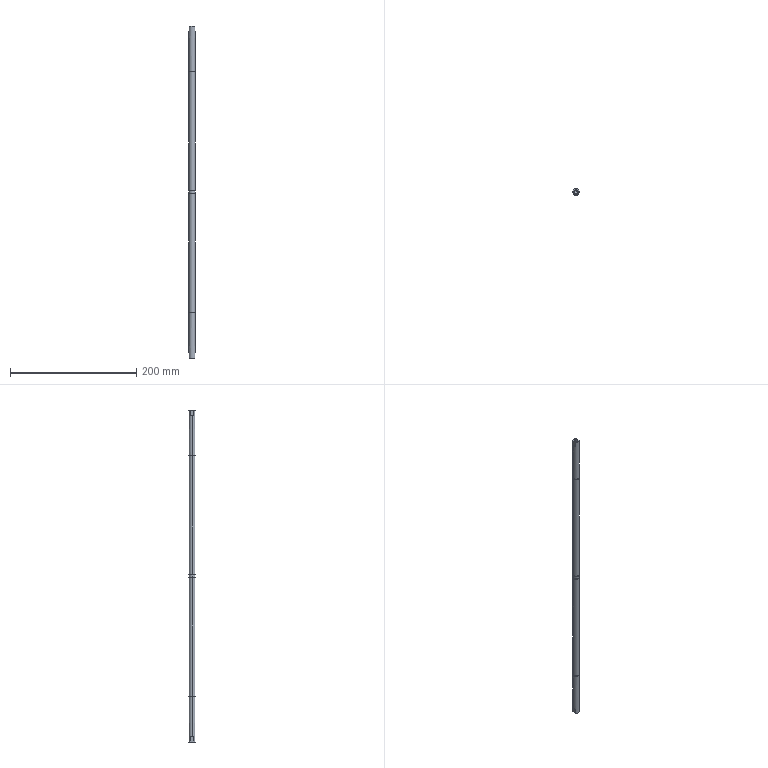Component | SolidWorks | RollerAxis2-1 | 1 solid | 48 faces | box 10 x 10 x 525 mm | volume 40269 mm3 | cylinder 22 | plane 18 | cone 8 | commonest cylinder face diameters 10 x10 9.65 x8 5 x4
build123d program:
from build123d import *

# Parameters (mm, degrees)
CUT_EXTRUDE1_START                 = -8
CUT_EXTRUDE1_DEPTH                 = 8
CUT_EXTRUDE2_START                 = -8
CUT_EXTRUDE2_DEPTH                 = 8
CUT_EXTRUDE3_DEPTH                 = 8
CUT_EXTRUDE4_DEPTH                 = 8
F_5_0_5_DIAMETER_HOLE1_D           = 5
F_5_0_5_DIAMETER_HOLE1_DEPTH       = 20
F_5_0_5_DIAMETER_HOLE1_CSINK_D     = 6.05
F_5_0_5_DIAMETER_HOLE1_CSINK_ANGLE = 90
F_5_0_5_DIAMETER_HOLE1_TIP         = 1.502
F_5_0_5_DIAMETER_HOLE2_D           = 5
F_5_0_5_DIAMETER_HOLE2_DEPTH       = 20
F_5_0_5_DIAMETER_HOLE2_CSINK_D     = 6.05
F_5_0_5_DIAMETER_HOLE2_CSINK_ANGLE = 90
F_5_0_5_DIAMETER_HOLE2_TIP         = 1.502


with BuildPart() as part:
    # Sketch1 → Revolve1 (revolve)
    with BuildSketch(Plane(origin=(0, 0, 0), x_dir=(-1, 0, 0), z_dir=(0, 0, -1)), mode=Mode.PRIVATE) as revolve1_sk:
        Polygon((-262.5, 5), (-262.5, 0), (262.5, 0), (262.5, 5), (191.1, 5), (191.1, 4.825), (190, 4.825), (190, 5), (3, 5), (3, 4.825), (1.9, 4.825), (1.9, 5), (-1.9, 5), (-1.9, 4.825), (-3, 4.825), (-3, 5), (-190, 5), (-190, 4.825), (-191.1, 4.825), (-191.1, 5), align=None)
    revolve(revolve1_sk.sketch.rotate(Axis((262.5, 0, 0), (-1, 0, 0)), 270), axis=Axis((262.5, 0, 0), (-1, 0, 0)))

    # Sketch2 → Cut-Extrude1 (cut)
    with BuildSketch(Plane.ZY.offset(262.5).offset(CUT_EXTRUDE1_START)):
        with BuildLine():
            Line((-4, -3), (-4, 3))
            ThreePointArc((-4, 3), (-5, 0), (-4, -3))
        make_face()
    extrude(amount=CUT_EXTRUDE1_DEPTH, mode=Mode.SUBTRACT)

    # Sketch3 → Cut-Extrude2 (cut)
    with BuildSketch(Plane.ZY.offset(262.5).offset(CUT_EXTRUDE2_START)):
        with BuildLine():
            Line((4, 3), (4, -3))
            ThreePointArc((4, -3), (5, 0), (4, 3))
        make_face()
    extrude(amount=CUT_EXTRUDE2_DEPTH, mode=Mode.SUBTRACT)

    # Sketch4 → Cut-Extrude3 (cut)
    with BuildSketch(Plane(origin=(262.5, 0, 0), x_dir=(0, 0, -1), z_dir=(1, 0, 0))):
        with BuildLine():
            Line((4, 3), (4, -3))
            ThreePointArc((4, -3), (5, 0), (4, 3))
        make_face()
    extrude(amount=-CUT_EXTRUDE3_DEPTH, mode=Mode.SUBTRACT)

    # Sketch5 → Cut-Extrude4 (cut)
    with BuildSketch(Plane(origin=(262.5, 0, 0), x_dir=(0, 0, -1), z_dir=(1, 0, 0))):
        with BuildLine():
            Line((-4, -3), (-4, 3))
            ThreePointArc((-4, 3), (-5, 0), (-4, -3))
        make_face()
    extrude(amount=-CUT_EXTRUDE4_DEPTH, mode=Mode.SUBTRACT)

    # 5.0 _5_ Diameter Hole1
    with Locations(Plane(origin=(262.5, 0, 0), x_dir=(0, 0, -1), z_dir=(1, 0, 0))):
        with Locations((0, 0)):
            CounterSinkHole(F_5_0_5_DIAMETER_HOLE1_D / 2, F_5_0_5_DIAMETER_HOLE1_CSINK_D / 2, depth=F_5_0_5_DIAMETER_HOLE1_DEPTH, counter_sink_angle=F_5_0_5_DIAMETER_HOLE1_CSINK_ANGLE)
            with Locations((0, 0, -(F_5_0_5_DIAMETER_HOLE1_DEPTH + F_5_0_5_DIAMETER_HOLE1_TIP / 2))):  # 118° drill point
                Cone(0, F_5_0_5_DIAMETER_HOLE1_D / 2, F_5_0_5_DIAMETER_HOLE1_TIP, mode=Mode.SUBTRACT)

    # 5.0 _5_ Diameter Hole2
    with Locations(Plane.ZY.offset(262.5)):
        with Locations((0, 0)):
            CounterSinkHole(F_5_0_5_DIAMETER_HOLE2_D / 2, F_5_0_5_DIAMETER_HOLE2_CSINK_D / 2, depth=F_5_0_5_DIAMETER_HOLE2_DEPTH, counter_sink_angle=F_5_0_5_DIAMETER_HOLE2_CSINK_ANGLE)
            with Locations((0, 0, -(F_5_0_5_DIAMETER_HOLE2_DEPTH + F_5_0_5_DIAMETER_HOLE2_TIP / 2))):  # 118° drill point
                Cone(0, F_5_0_5_DIAMETER_HOLE2_D / 2, F_5_0_5_DIAMETER_HOLE2_TIP, mode=Mode.SUBTRACT)


solid = part.part

# Placed as in the assembly
solid = solid.moved(Location((-66, -158, 0), (0, 90, 0)))